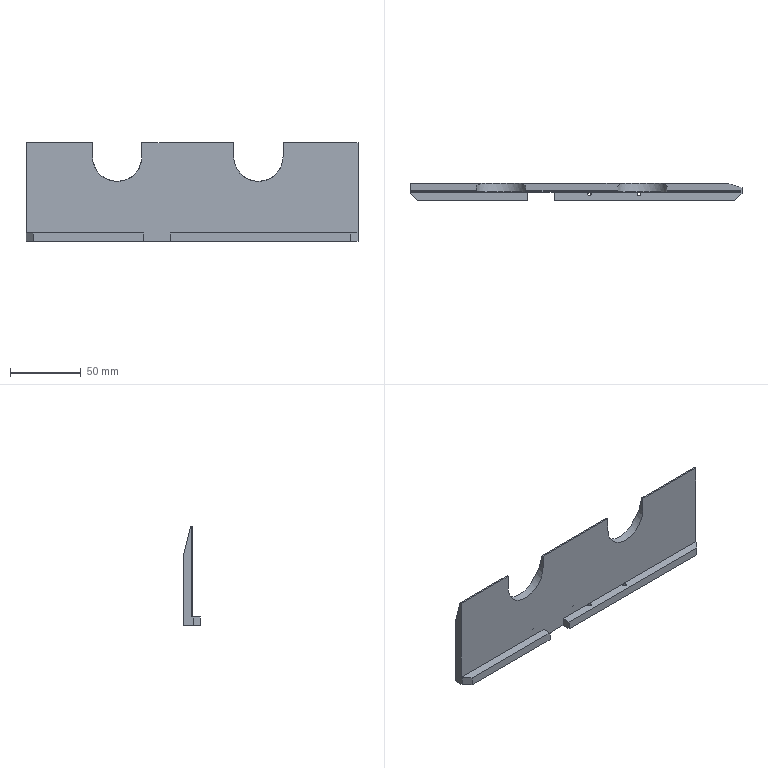Component | SolidWorks | P-SLJ-002-2_P-SLJ-002-003-1 | 1 solid | 38 faces | box 235 x 12 x 70 mm | volume 87007 mm3 | plane 24 | cylinder 10 | cone 4 | commonest cylinder face diameters 3.3 x4 2.5 x4 35 x2 | material A3
build123d program:
from build123d import *

# Parameters (mm, degrees)
EXTRUDE1_DEPTH        = 117.5
EXTRUDE2_REACH        = 247.497
EXTRUDE3_DEPTH        = 138.296
M3_TAPPED_HOLE1_D     = 2.5
M3_TAPPED_HOLE1_DEPTH = 8.5
M3_TAPPED_HOLE1_TIP   = 0.7511
M4_TAPPED_HOLE1_D     = 3.3
M4_TAPPED_HOLE1_DEPTH = 11.5
M4_TAPPED_HOLE1_TIP   = 0.9914
SKETCH9_W             = 19
SKETCH9_H             = 6
EXTRUDE4_DEPTH        = 138.296
CHAMFER1_SIZE         = 5
CHAMFER1_2_SIZE       = 10
CHAMFER1_2_SIZE2      = 3


with BuildPart() as part:
    # Sketch1 → Extrude1 (new, symmetric)
    with BuildSketch(Plane(origin=(0, 0, 0), x_dir=(0, 0, -1), z_dir=(1, 0, 0))):
        Polygon((0, 0), (-6, 0), (-6, 6), (-70, 6), (-70, 12), (0, 12), align=None)
    extrude(amount=EXTRUDE1_DEPTH, both=True)

    # Sketch2 → Extrude2 (cut, up to next)
    with BuildSketch(Plane(origin=(117.5, 0, 0), x_dir=(0, 0, -1), z_dir=(1, 0, 0)), mode=Mode.PRIVATE) as extrude2_sk1:
        Polygon((-70, 7), (-70, 12), (-50, 12), align=None)
    extrude2_tool1 = extrude(extrude2_sk1.sketch, amount=-EXTRUDE2_REACH, mode=Mode.PRIVATE) & part.part
    add(extrude2_tool1.solids().sort_by_distance((117.5, 10.333, 63.333))[0], mode=Mode.SUBTRACT)

    # Sketch3 → Extrude3 (cut, through all)
    with BuildSketch(Plane(origin=(0, 12, 0), x_dir=(1, 0, 0), z_dir=(0, 1, 0))):
        with BuildLine():
            Line((-70.5, -60), (-70.5, -70))
            Line((-70.5, -70), (-35.5, -70))
            Line((-35.5, -70), (-35.5, -60))
            ThreePointArc((-35.5, -60), (-53, -42.5), (-70.5, -60))
        make_face()
        with BuildLine():
            Line((29.5, -60), (29.5, -70))
            Line((29.5, -70), (64.5, -70))
            Line((64.5, -70), (64.5, -60))
            ThreePointArc((64.5, -60), (47, -42.5), (29.5, -60))
        make_face()
    extrude(amount=-EXTRUDE3_DEPTH, mode=Mode.SUBTRACT)

    # M3 Tapped Hole1
    with Locations(Plane(origin=(0, 0, 0), x_dir=(-1, 0, 0), z_dir=(0, 0, -1))):
        with Locations((-44.5, 4.5), (-9.5, 4.5)):
            Hole(M3_TAPPED_HOLE1_D / 2, depth=M3_TAPPED_HOLE1_DEPTH)
            with Locations((0, 0, -(M3_TAPPED_HOLE1_DEPTH + M3_TAPPED_HOLE1_TIP / 2))):  # 118° drill point
                Cone(0, M3_TAPPED_HOLE1_D / 2, M3_TAPPED_HOLE1_TIP, mode=Mode.SUBTRACT)

    # M4 Tapped Hole1
    with Locations(Plane(origin=(0, 0, 0), x_dir=(-1, 0, 0), z_dir=(0, 0, -1))):
        with Locations((5, 8), (45, 8)):
            Hole(M4_TAPPED_HOLE1_D / 2, depth=M4_TAPPED_HOLE1_DEPTH)
            with Locations((0, 0, -(M4_TAPPED_HOLE1_DEPTH + M4_TAPPED_HOLE1_TIP / 2))):  # 118° drill point
                Cone(0, M4_TAPPED_HOLE1_D / 2, M4_TAPPED_HOLE1_TIP, mode=Mode.SUBTRACT)

    # Sketch9 → Extrude4 (cut, through all)
    with BuildSketch(Plane(origin=(0, 0, 0), x_dir=(-1, 0, 0), z_dir=(0, 0, -1))):
        with Locations((25, 3)):
            Rectangle(SKETCH9_W, SKETCH9_H)
    extrude(amount=-EXTRUDE4_DEPTH, mode=Mode.SUBTRACT)

    # Chamfer1
    chamfer1_edges = [part.edges().sort_by_distance(p)[0] for p in [
        (117.5, 0, 3),
        (-117.5, 0, 3),
    ]]
    chamfer(chamfer1_edges, length=CHAMFER1_SIZE)

    # Chamfer1_2
    chamfer1_2_edges = [part.edges().sort_by_distance(p)[0] for p in [
        (117.5, 12, 25),
    ]]
    chamfer1_2_side = [part.faces().sort_by_distance(p)[0] for p in [
        (0.07923, 12, 24.421),
    ]]
    chamfer(chamfer1_2_edges, length=CHAMFER1_2_SIZE, length2=CHAMFER1_2_SIZE2, reference=chamfer1_2_side[0])


solid = part.part

# Placed as in the assembly
solid = solid.moved(Location((-220, -69, 928.634), (0, 0, 0)))